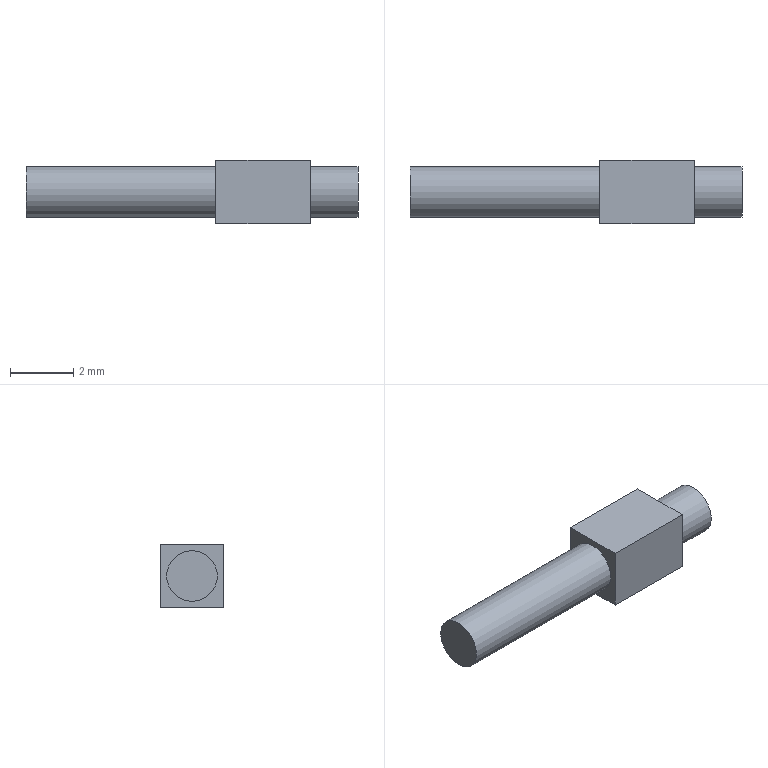Component | NX | MID_RECT_2_CIRC_2 | 1 solid | 10 faces | box 10.5 x 2 x 2 mm | volume 27 mm3 | plane 8 | cylinder 2 | commonest cylinder face diameters 1.6 x2
STEP:
#1=CARTESIAN_POINT('',(0.,0.,0.));
#2=DIRECTION('',(0.,0.,1.));
#3=DIRECTION('',(1.,0.,0.));
#4=AXIS2_PLACEMENT_3D('',#1,#2,#3);
#5=CARTESIAN_POINT('',(15.5,22.225,29.));
#6=VERTEX_POINT('',#5);
#7=CARTESIAN_POINT('',(18.5,22.225,29.));
#8=VERTEX_POINT('',#7);
#9=CARTESIAN_POINT('',(15.5,22.225,29.));
#10=DIRECTION('',(1.,-0.,0.));
#11=VECTOR('',#10,1.);
#12=LINE('',#9,#11);
#13=CARTESIAN_POINT('',(15.5,22.225,31.));
#14=DIRECTION('',(0.,1.,0.));
#15=DIRECTION('',(-1.,0.,0.));
#16=AXIS2_PLACEMENT_3D('',#13,#14,#15);
#17=PLANE('',#16);
#18=CARTESIAN_POINT('',(0.,-2.));
#19=DIRECTION('',(-1.,0.));
#20=VECTOR('',#19,1.);
#21=LINE('',#18,#20);
#22=(GEOMETRIC_REPRESENTATION_CONTEXT(2)PARAMETRIC_REPRESENTATION_CONTEXT()REPRESENTATION_CONTEXT('',''));
#23=DEFINITIONAL_REPRESENTATION('',(#21),#22);
#24=PCURVE('',#17,#23);
#25=CARTESIAN_POINT('',(17.,23.225,29.));
#26=DIRECTION('',(0.,0.,1.));
#27=DIRECTION('',(1.,0.,0.));
#28=AXIS2_PLACEMENT_3D('',#25,#26,#27);
#29=PLANE('',#28);
#30=CARTESIAN_POINT('',(-1.5,-1.));
#31=DIRECTION('',(1.,-0.));
#32=VECTOR('',#31,1.);
#33=LINE('',#30,#32);
#34=(GEOMETRIC_REPRESENTATION_CONTEXT(2)PARAMETRIC_REPRESENTATION_CONTEXT()REPRESENTATION_CONTEXT('',''));
#35=DEFINITIONAL_REPRESENTATION('',(#33),#34);
#36=PCURVE('',#29,#35);
#37=SURFACE_CURVE('',#12,(#24,#36),.PCURVE_S1.);
#38=EDGE_CURVE('',#6,#8,#37,.T.);
#39=ORIENTED_EDGE('',*,*,#38,.T.);
#40=CARTESIAN_POINT('',(18.5,22.225,31.));
#41=VERTEX_POINT('',#40);
#42=CARTESIAN_POINT('',(18.5,22.225,31.));
#43=DIRECTION('',(0.,0.,-1.));
#44=VECTOR('',#43,1.);
#45=LINE('',#42,#44);
#46=CARTESIAN_POINT('',(-3.,0.));
#47=DIRECTION('',(0.,-1.));
#48=VECTOR('',#47,1.);
#49=LINE('',#46,#48);
#50=(GEOMETRIC_REPRESENTATION_CONTEXT(2)PARAMETRIC_REPRESENTATION_CONTEXT()REPRESENTATION_CONTEXT('',''));
#51=DEFINITIONAL_REPRESENTATION('',(#49),#50);
#52=PCURVE('',#17,#51);
#53=CARTESIAN_POINT('',(18.5,22.225,31.));
#54=DIRECTION('',(-1.,0.,0.));
#55=DIRECTION('',(0.,0.,1.));
#56=AXIS2_PLACEMENT_3D('',#53,#54,#55);
#57=PLANE('',#56);
#58=CARTESIAN_POINT('',(0.,0.));
#59=DIRECTION('',(-1.,0.));
#60=VECTOR('',#59,1.);
#61=LINE('',#58,#60);
#62=(GEOMETRIC_REPRESENTATION_CONTEXT(2)PARAMETRIC_REPRESENTATION_CONTEXT()REPRESENTATION_CONTEXT('',''));
#63=DEFINITIONAL_REPRESENTATION('',(#61),#62);
#64=PCURVE('',#57,#63);
#65=SURFACE_CURVE('',#45,(#52,#64),.PCURVE_S1.);
#66=EDGE_CURVE('',#41,#8,#65,.T.);
#67=ORIENTED_EDGE('',*,*,#66,.F.);
#68=CARTESIAN_POINT('',(15.5,22.225,31.));
#69=VERTEX_POINT('',#68);
#70=CARTESIAN_POINT('',(15.5,22.225,31.));
#71=DIRECTION('',(1.,-0.,0.));
#72=VECTOR('',#71,1.);
#73=LINE('',#70,#72);
#74=CARTESIAN_POINT('',(0.,0.));
#75=DIRECTION('',(-1.,0.));
#76=VECTOR('',#75,1.);
#77=LINE('',#74,#76);
#78=(GEOMETRIC_REPRESENTATION_CONTEXT(2)PARAMETRIC_REPRESENTATION_CONTEXT()REPRESENTATION_CONTEXT('',''));
#79=DEFINITIONAL_REPRESENTATION('',(#77),#78);
#80=PCURVE('',#17,#79);
#81=CARTESIAN_POINT('',(17.,23.225,31.));
#82=DIRECTION('',(0.,0.,1.));
#83=DIRECTION('',(1.,0.,0.));
#84=AXIS2_PLACEMENT_3D('',#81,#82,#83);
#85=PLANE('',#84);
#86=CARTESIAN_POINT('',(-1.5,-1.));
#87=DIRECTION('',(1.,-0.));
#88=VECTOR('',#87,1.);
#89=LINE('',#86,#88);
#90=(GEOMETRIC_REPRESENTATION_CONTEXT(2)PARAMETRIC_REPRESENTATION_CONTEXT()REPRESENTATION_CONTEXT('',''));
#91=DEFINITIONAL_REPRESENTATION('',(#89),#90);
#92=PCURVE('',#85,#91);
#93=SURFACE_CURVE('',#73,(#80,#92),.PCURVE_S1.);
#94=EDGE_CURVE('',#69,#41,#93,.T.);
#95=ORIENTED_EDGE('',*,*,#94,.F.);
#96=CARTESIAN_POINT('',(15.5,22.225,31.));
#97=DIRECTION('',(0.,0.,-1.));
#98=VECTOR('',#97,1.);
#99=LINE('',#96,#98);
#100=CARTESIAN_POINT('',(0.,0.));
#101=DIRECTION('',(0.,-1.));
#102=VECTOR('',#101,1.);
#103=LINE('',#100,#102);
#104=(GEOMETRIC_REPRESENTATION_CONTEXT(2)PARAMETRIC_REPRESENTATION_CONTEXT()REPRESENTATION_CONTEXT('',''));
#105=DEFINITIONAL_REPRESENTATION('',(#103),#104);
#106=PCURVE('',#17,#105);
#107=CARTESIAN_POINT('',(15.5,24.225,31.));
#108=DIRECTION('',(1.,0.,0.));
#109=DIRECTION('',(0.,0.,-1.));
#110=AXIS2_PLACEMENT_3D('',#107,#108,#109);
#111=PLANE('',#110);
#112=CARTESIAN_POINT('',(0.,-2.));
#113=DIRECTION('',(1.,0.));
#114=VECTOR('',#113,1.);
#115=LINE('',#112,#114);
#116=(GEOMETRIC_REPRESENTATION_CONTEXT(2)PARAMETRIC_REPRESENTATION_CONTEXT()REPRESENTATION_CONTEXT('',''));
#117=DEFINITIONAL_REPRESENTATION('',(#115),#116);
#118=PCURVE('',#111,#117);
#119=SURFACE_CURVE('',#99,(#106,#118),.PCURVE_S1.);
#120=EDGE_CURVE('',#69,#6,#119,.T.);
#121=ORIENTED_EDGE('',*,*,#120,.T.);
#122=EDGE_LOOP('',(#39,#67,#95,#121));
#123=FACE_BOUND('',#122,.T.);
#124=ADVANCED_FACE('',(#123),#17,.F.);
#125=CARTESIAN_POINT('',(18.5,23.225,30.8));
#126=VERTEX_POINT('',#125);
#127=CARTESIAN_POINT('',(18.5,23.225,30.));
#128=DIRECTION('',(1.,0.,0.));
#129=DIRECTION('',(0.,0.,1.));
#130=AXIS2_PLACEMENT_3D('',#127,#128,#129);
#131=CIRCLE('',#130,0.8);
#132=CARTESIAN_POINT('',(-0.2,1.));
#133=CARTESIAN_POINT('',(-0.2,-0.3856));
#134=CARTESIAN_POINT('',(-1.4,0.3072));
#135=CARTESIAN_POINT('',(-2.6,1.));
#136=CARTESIAN_POINT('',(-1.4,1.693));
#137=CARTESIAN_POINT('',(-0.2,2.386));
#138=CARTESIAN_POINT('',(-0.2,1.));
#139=(BOUNDED_CURVE()B_SPLINE_CURVE(2,(#132,#133,#134,#135,#136,#137,#138),.UNSPECIFIED.,.T.,.F.)B_SPLINE_CURVE_WITH_KNOTS((1,2,2,2,2,1),(-2.094,0.,2.094,4.189,6.283,8.378),.UNSPECIFIED.)CURVE()GEOMETRIC_REPRESENTATION_ITEM()RATIONAL_B_SPLINE_CURVE((1.,0.5,1.,0.5,1.,0.5,1.))REPRESENTATION_ITEM(''));
#140=(GEOMETRIC_REPRESENTATION_CONTEXT(2)PARAMETRIC_REPRESENTATION_CONTEXT()REPRESENTATION_CONTEXT('',''));
#141=DEFINITIONAL_REPRESENTATION('',(#139),#140);
#142=PCURVE('',#57,#141);
#143=CARTESIAN_POINT('',(9.5,23.225,30.));
#144=DIRECTION('',(1.,0.,0.));
#145=DIRECTION('',(0.,0.,-1.));
#146=AXIS2_PLACEMENT_3D('',#143,#144,#145);
#147=CYLINDRICAL_SURFACE('',#146,0.8);
#148=CARTESIAN_POINT('',(3.142,9.));
#149=DIRECTION('',(1.,0.));
#150=VECTOR('',#149,1.);
#151=LINE('',#148,#150);
#152=(GEOMETRIC_REPRESENTATION_CONTEXT(2)PARAMETRIC_REPRESENTATION_CONTEXT()REPRESENTATION_CONTEXT('',''));
#153=DEFINITIONAL_REPRESENTATION('',(#151),#152);
#154=PCURVE('',#147,#153);
#155=SURFACE_CURVE('',#131,(#142,#154),.PCURVE_S1.);
#156=EDGE_CURVE('',#126,#126,#155,.T.);
#157=ORIENTED_EDGE('',*,*,#156,.F.);
#158=EDGE_LOOP('',(#157));
#159=FACE_BOUND('',#158,.T.);
#160=CARTESIAN_POINT('',(18.5,24.225,29.));
#161=VERTEX_POINT('',#160);
#162=CARTESIAN_POINT('',(18.5,22.225,29.));
#163=DIRECTION('',(0.,1.,0.));
#164=VECTOR('',#163,1.);
#165=LINE('',#162,#164);
#166=CARTESIAN_POINT('',(-2.,0.));
#167=DIRECTION('',(0.,1.));
#168=VECTOR('',#167,1.);
#169=LINE('',#166,#168);
#170=(GEOMETRIC_REPRESENTATION_CONTEXT(2)PARAMETRIC_REPRESENTATION_CONTEXT()REPRESENTATION_CONTEXT('',''));
#171=DEFINITIONAL_REPRESENTATION('',(#169),#170);
#172=PCURVE('',#57,#171);
#173=CARTESIAN_POINT('',(1.5,-1.));
#174=DIRECTION('',(0.,1.));
#175=VECTOR('',#174,1.);
#176=LINE('',#173,#175);
#177=(GEOMETRIC_REPRESENTATION_CONTEXT(2)PARAMETRIC_REPRESENTATION_CONTEXT()REPRESENTATION_CONTEXT('',''));
#178=DEFINITIONAL_REPRESENTATION('',(#176),#177);
#179=PCURVE('',#29,#178);
#180=SURFACE_CURVE('',#165,(#172,#179),.PCURVE_S1.);
#181=EDGE_CURVE('',#8,#161,#180,.T.);
#182=ORIENTED_EDGE('',*,*,#181,.T.);
#183=CARTESIAN_POINT('',(18.5,24.225,31.));
#184=VERTEX_POINT('',#183);
#185=CARTESIAN_POINT('',(18.5,24.225,31.));
#186=DIRECTION('',(0.,0.,-1.));
#187=VECTOR('',#186,1.);
#188=LINE('',#185,#187);
#189=CARTESIAN_POINT('',(0.,2.));
#190=DIRECTION('',(-1.,0.));
#191=VECTOR('',#190,1.);
#192=LINE('',#189,#191);
#193=(GEOMETRIC_REPRESENTATION_CONTEXT(2)PARAMETRIC_REPRESENTATION_CONTEXT()REPRESENTATION_CONTEXT('',''));
#194=DEFINITIONAL_REPRESENTATION('',(#192),#193);
#195=PCURVE('',#57,#194);
#196=CARTESIAN_POINT('',(18.5,24.225,31.));
#197=DIRECTION('',(-0.,-1.,0.));
#198=DIRECTION('',(1.,-0.,0.));
#199=AXIS2_PLACEMENT_3D('',#196,#197,#198);
#200=PLANE('',#199);
#201=CARTESIAN_POINT('',(0.,0.));
#202=DIRECTION('',(0.,-1.));
#203=VECTOR('',#202,1.);
#204=LINE('',#201,#203);
#205=(GEOMETRIC_REPRESENTATION_CONTEXT(2)PARAMETRIC_REPRESENTATION_CONTEXT()REPRESENTATION_CONTEXT('',''));
#206=DEFINITIONAL_REPRESENTATION('',(#204),#205);
#207=PCURVE('',#200,#206);
#208=SURFACE_CURVE('',#188,(#195,#207),.PCURVE_S1.);
#209=EDGE_CURVE('',#184,#161,#208,.T.);
#210=ORIENTED_EDGE('',*,*,#209,.F.);
#211=CARTESIAN_POINT('',(18.5,22.225,31.));
#212=DIRECTION('',(0.,1.,0.));
#213=VECTOR('',#212,1.);
#214=LINE('',#211,#213);
#215=CARTESIAN_POINT('',(0.,0.));
#216=DIRECTION('',(0.,1.));
#217=VECTOR('',#216,1.);
#218=LINE('',#215,#217);
#219=(GEOMETRIC_REPRESENTATION_CONTEXT(2)PARAMETRIC_REPRESENTATION_CONTEXT()REPRESENTATION_CONTEXT('',''));
#220=DEFINITIONAL_REPRESENTATION('',(#218),#219);
#221=PCURVE('',#57,#220);
#222=CARTESIAN_POINT('',(1.5,-1.));
#223=DIRECTION('',(0.,1.));
#224=VECTOR('',#223,1.);
#225=LINE('',#222,#224);
#226=(GEOMETRIC_REPRESENTATION_CONTEXT(2)PARAMETRIC_REPRESENTATION_CONTEXT()REPRESENTATION_CONTEXT('',''));
#227=DEFINITIONAL_REPRESENTATION('',(#225),#226);
#228=PCURVE('',#85,#227);
#229=SURFACE_CURVE('',#214,(#221,#228),.PCURVE_S1.);
#230=EDGE_CURVE('',#41,#184,#229,.T.);
#231=ORIENTED_EDGE('',*,*,#230,.F.);
#232=ORIENTED_EDGE('',*,*,#66,.T.);
#233=EDGE_LOOP('',(#182,#210,#231,#232));
#234=FACE_BOUND('',#233,.T.);
#235=ADVANCED_FACE('',(#159,#234),#57,.F.);
#236=CARTESIAN_POINT('',(15.5,24.225,29.));
#237=VERTEX_POINT('',#236);
#238=CARTESIAN_POINT('',(18.5,24.225,29.));
#239=DIRECTION('',(-1.,0.,0.));
#240=VECTOR('',#239,1.);
#241=LINE('',#238,#240);
#242=CARTESIAN_POINT('',(0.,-2.));
#243=DIRECTION('',(-1.,0.));
#244=VECTOR('',#243,1.);
#245=LINE('',#242,#244);
#246=(GEOMETRIC_REPRESENTATION_CONTEXT(2)PARAMETRIC_REPRESENTATION_CONTEXT()REPRESENTATION_CONTEXT('',''));
#247=DEFINITIONAL_REPRESENTATION('',(#245),#246);
#248=PCURVE('',#200,#247);
#249=CARTESIAN_POINT('',(1.5,1.));
#250=DIRECTION('',(-1.,0.));
#251=VECTOR('',#250,1.);
#252=LINE('',#249,#251);
#253=(GEOMETRIC_REPRESENTATION_CONTEXT(2)PARAMETRIC_REPRESENTATION_CONTEXT()REPRESENTATION_CONTEXT('',''));
#254=DEFINITIONAL_REPRESENTATION('',(#252),#253);
#255=PCURVE('',#29,#254);
#256=SURFACE_CURVE('',#241,(#248,#255),.PCURVE_S1.);
#257=EDGE_CURVE('',#161,#237,#256,.T.);
#258=ORIENTED_EDGE('',*,*,#257,.T.);
#259=CARTESIAN_POINT('',(15.5,24.225,31.));
#260=VERTEX_POINT('',#259);
#261=CARTESIAN_POINT('',(15.5,24.225,31.));
#262=DIRECTION('',(0.,0.,-1.));
#263=VECTOR('',#262,1.);
#264=LINE('',#261,#263);
#265=CARTESIAN_POINT('',(-3.,0.));
#266=DIRECTION('',(0.,-1.));
#267=VECTOR('',#266,1.);
#268=LINE('',#265,#267);
#269=(GEOMETRIC_REPRESENTATION_CONTEXT(2)PARAMETRIC_REPRESENTATION_CONTEXT()REPRESENTATION_CONTEXT('',''));
#270=DEFINITIONAL_REPRESENTATION('',(#268),#269);
#271=PCURVE('',#200,#270);
#272=CARTESIAN_POINT('',(0.,0.));
#273=DIRECTION('',(1.,0.));
#274=VECTOR('',#273,1.);
#275=LINE('',#272,#274);
#276=(GEOMETRIC_REPRESENTATION_CONTEXT(2)PARAMETRIC_REPRESENTATION_CONTEXT()REPRESENTATION_CONTEXT('',''));
#277=DEFINITIONAL_REPRESENTATION('',(#275),#276);
#278=PCURVE('',#111,#277);
#279=SURFACE_CURVE('',#264,(#271,#278),.PCURVE_S1.);
#280=EDGE_CURVE('',#260,#237,#279,.T.);
#281=ORIENTED_EDGE('',*,*,#280,.F.);
#282=CARTESIAN_POINT('',(18.5,24.225,31.));
#283=DIRECTION('',(-1.,0.,0.));
#284=VECTOR('',#283,1.);
#285=LINE('',#282,#284);
#286=CARTESIAN_POINT('',(0.,0.));
#287=DIRECTION('',(-1.,0.));
#288=VECTOR('',#287,1.);
#289=LINE('',#286,#288);
#290=(GEOMETRIC_REPRESENTATION_CONTEXT(2)PARAMETRIC_REPRESENTATION_CONTEXT()REPRESENTATION_CONTEXT('',''));
#291=DEFINITIONAL_REPRESENTATION('',(#289),#290);
#292=PCURVE('',#200,#291);
#293=CARTESIAN_POINT('',(1.5,1.));
#294=DIRECTION('',(-1.,0.));
#295=VECTOR('',#294,1.);
#296=LINE('',#293,#295);
#297=(GEOMETRIC_REPRESENTATION_CONTEXT(2)PARAMETRIC_REPRESENTATION_CONTEXT()REPRESENTATION_CONTEXT('',''));
#298=DEFINITIONAL_REPRESENTATION('',(#296),#297);
#299=PCURVE('',#85,#298);
#300=SURFACE_CURVE('',#285,(#292,#299),.PCURVE_S1.);
#301=EDGE_CURVE('',#184,#260,#300,.T.);
#302=ORIENTED_EDGE('',*,*,#301,.F.);
#303=ORIENTED_EDGE('',*,*,#209,.T.);
#304=EDGE_LOOP('',(#258,#281,#302,#303));
#305=FACE_BOUND('',#304,.T.);
#306=ADVANCED_FACE('',(#305),#200,.F.);
#307=CARTESIAN_POINT('',(15.5,23.225,29.2));
#308=VERTEX_POINT('',#307);
#309=CARTESIAN_POINT('',(15.5,23.225,30.));
#310=DIRECTION('',(-1.,0.,0.));
#311=DIRECTION('',(0.,0.,-1.));
#312=AXIS2_PLACEMENT_3D('',#309,#310,#311);
#313=CIRCLE('',#312,0.8);
#314=CARTESIAN_POINT('',(1.8,-1.));
#315=CARTESIAN_POINT('',(1.8,-2.386));
#316=CARTESIAN_POINT('',(0.6,-1.693));
#317=CARTESIAN_POINT('',(-0.6,-1.));
#318=CARTESIAN_POINT('',(0.6,-0.3072));
#319=CARTESIAN_POINT('',(1.8,0.3856));
#320=CARTESIAN_POINT('',(1.8,-1.));
#321=(BOUNDED_CURVE()B_SPLINE_CURVE(2,(#314,#315,#316,#317,#318,#319,#320),.UNSPECIFIED.,.T.,.F.)B_SPLINE_CURVE_WITH_KNOTS((1,2,2,2,2,1),(-2.094,0.,2.094,4.189,6.283,8.378),.UNSPECIFIED.)CURVE()GEOMETRIC_REPRESENTATION_ITEM()RATIONAL_B_SPLINE_CURVE((1.,0.5,1.,0.5,1.,0.5,1.))REPRESENTATION_ITEM(''));
#322=(GEOMETRIC_REPRESENTATION_CONTEXT(2)PARAMETRIC_REPRESENTATION_CONTEXT()REPRESENTATION_CONTEXT('',''));
#323=DEFINITIONAL_REPRESENTATION('',(#321),#322);
#324=PCURVE('',#111,#323);
#325=CARTESIAN_POINT('',(9.5,23.225,30.));
#326=DIRECTION('',(1.,0.,0.));
#327=DIRECTION('',(0.,0.,-1.));
#328=AXIS2_PLACEMENT_3D('',#325,#326,#327);
#329=CYLINDRICAL_SURFACE('',#328,0.8);
#330=CARTESIAN_POINT('',(6.283,6.));
#331=DIRECTION('',(-1.,0.));
#332=VECTOR('',#331,1.);
#333=LINE('',#330,#332);
#334=(GEOMETRIC_REPRESENTATION_CONTEXT(2)PARAMETRIC_REPRESENTATION_CONTEXT()REPRESENTATION_CONTEXT('',''));
#335=DEFINITIONAL_REPRESENTATION('',(#333),#334);
#336=PCURVE('',#329,#335);
#337=SURFACE_CURVE('',#313,(#324,#336),.PCURVE_S1.);
#338=EDGE_CURVE('',#308,#308,#337,.T.);
#339=ORIENTED_EDGE('',*,*,#338,.F.);
#340=EDGE_LOOP('',(#339));
#341=FACE_BOUND('',#340,.T.);
#342=CARTESIAN_POINT('',(15.5,24.225,29.));
#343=DIRECTION('',(0.,-1.,0.));
#344=VECTOR('',#343,1.);
#345=LINE('',#342,#344);
#346=CARTESIAN_POINT('',(2.,0.));
#347=DIRECTION('',(0.,-1.));
#348=VECTOR('',#347,1.);
#349=LINE('',#346,#348);
#350=(GEOMETRIC_REPRESENTATION_CONTEXT(2)PARAMETRIC_REPRESENTATION_CONTEXT()REPRESENTATION_CONTEXT('',''));
#351=DEFINITIONAL_REPRESENTATION('',(#349),#350);
#352=PCURVE('',#111,#351);
#353=CARTESIAN_POINT('',(-1.5,1.));
#354=DIRECTION('',(0.,-1.));
#355=VECTOR('',#354,1.);
#356=LINE('',#353,#355);
#357=(GEOMETRIC_REPRESENTATION_CONTEXT(2)PARAMETRIC_REPRESENTATION_CONTEXT()REPRESENTATION_CONTEXT('',''));
#358=DEFINITIONAL_REPRESENTATION('',(#356),#357);
#359=PCURVE('',#29,#358);
#360=SURFACE_CURVE('',#345,(#352,#359),.PCURVE_S1.);
#361=EDGE_CURVE('',#237,#6,#360,.T.);
#362=ORIENTED_EDGE('',*,*,#361,.T.);
#363=ORIENTED_EDGE('',*,*,#120,.F.);
#364=CARTESIAN_POINT('',(15.5,24.225,31.));
#365=DIRECTION('',(0.,-1.,0.));
#366=VECTOR('',#365,1.);
#367=LINE('',#364,#366);
#368=CARTESIAN_POINT('',(0.,0.));
#369=DIRECTION('',(0.,-1.));
#370=VECTOR('',#369,1.);
#371=LINE('',#368,#370);
#372=(GEOMETRIC_REPRESENTATION_CONTEXT(2)PARAMETRIC_REPRESENTATION_CONTEXT()REPRESENTATION_CONTEXT('',''));
#373=DEFINITIONAL_REPRESENTATION('',(#371),#372);
#374=PCURVE('',#111,#373);
#375=CARTESIAN_POINT('',(-1.5,1.));
#376=DIRECTION('',(0.,-1.));
#377=VECTOR('',#376,1.);
#378=LINE('',#375,#377);
#379=(GEOMETRIC_REPRESENTATION_CONTEXT(2)PARAMETRIC_REPRESENTATION_CONTEXT()REPRESENTATION_CONTEXT('',''));
#380=DEFINITIONAL_REPRESENTATION('',(#378),#379);
#381=PCURVE('',#85,#380);
#382=SURFACE_CURVE('',#367,(#374,#381),.PCURVE_S1.);
#383=EDGE_CURVE('',#260,#69,#382,.T.);
#384=ORIENTED_EDGE('',*,*,#383,.F.);
#385=ORIENTED_EDGE('',*,*,#280,.T.);
#386=EDGE_LOOP('',(#362,#363,#384,#385));
#387=FACE_BOUND('',#386,.T.);
#388=ADVANCED_FACE('',(#341,#387),#111,.F.);
#389=ORIENTED_EDGE('',*,*,#94,.T.);
#390=ORIENTED_EDGE('',*,*,#230,.T.);
#391=ORIENTED_EDGE('',*,*,#301,.T.);
#392=ORIENTED_EDGE('',*,*,#383,.T.);
#393=EDGE_LOOP('',(#389,#390,#391,#392));
#394=FACE_BOUND('',#393,.T.);
#395=ADVANCED_FACE('',(#394),#85,.T.);
#396=ORIENTED_EDGE('',*,*,#38,.F.);
#397=ORIENTED_EDGE('',*,*,#361,.F.);
#398=ORIENTED_EDGE('',*,*,#257,.F.);
#399=ORIENTED_EDGE('',*,*,#181,.F.);
#400=EDGE_LOOP('',(#396,#397,#398,#399));
#401=FACE_BOUND('',#400,.T.);
#402=ADVANCED_FACE('',(#401),#29,.F.);
#403=CARTESIAN_POINT('',(9.5,23.225,30.8));
#404=VERTEX_POINT('',#403);
#405=CARTESIAN_POINT('',(9.5,23.225,29.2));
#406=VERTEX_POINT('',#405);
#407=CARTESIAN_POINT('',(9.5,23.225,30.));
#408=DIRECTION('',(-1.,0.,0.));
#409=DIRECTION('',(0.,0.,1.));
#410=AXIS2_PLACEMENT_3D('',#407,#408,#409);
#411=CIRCLE('',#410,0.8);
#412=CARTESIAN_POINT('',(9.5,23.225,30.));
#413=DIRECTION('',(-1.,0.,0.));
#414=DIRECTION('',(0.,0.,1.));
#415=AXIS2_PLACEMENT_3D('',#412,#413,#414);
#416=PLANE('',#415);
#417=CARTESIAN_POINT('',(0.,0.));
#418=DIRECTION('',(1.,0.));
#419=AXIS2_PLACEMENT_2D('',#417,#418);
#420=CIRCLE('',#419,0.8);
#421=(GEOMETRIC_REPRESENTATION_CONTEXT(2)PARAMETRIC_REPRESENTATION_CONTEXT()REPRESENTATION_CONTEXT('',''));
#422=DEFINITIONAL_REPRESENTATION('',(#420),#421);
#423=PCURVE('',#416,#422);
#424=CARTESIAN_POINT('',(3.142,0.));
#425=DIRECTION('',(-1.,0.));
#426=VECTOR('',#425,1.);
#427=LINE('',#424,#426);
#428=(GEOMETRIC_REPRESENTATION_CONTEXT(2)PARAMETRIC_REPRESENTATION_CONTEXT()REPRESENTATION_CONTEXT('',''));
#429=DEFINITIONAL_REPRESENTATION('',(#427),#428);
#430=PCURVE('',#329,#429);
#431=SURFACE_CURVE('',#411,(#423,#430),.PCURVE_S1.);
#432=EDGE_CURVE('',#404,#406,#431,.T.);
#433=ORIENTED_EDGE('',*,*,#432,.T.);
#434=CARTESIAN_POINT('',(9.5,23.225,30.));
#435=DIRECTION('',(-1.,0.,0.));
#436=DIRECTION('',(0.,0.,1.));
#437=AXIS2_PLACEMENT_3D('',#434,#435,#436);
#438=CIRCLE('',#437,0.8);
#439=CARTESIAN_POINT('',(0.,0.));
#440=DIRECTION('',(1.,0.));
#441=AXIS2_PLACEMENT_2D('',#439,#440);
#442=CIRCLE('',#441,0.8);
#443=(GEOMETRIC_REPRESENTATION_CONTEXT(2)PARAMETRIC_REPRESENTATION_CONTEXT()REPRESENTATION_CONTEXT('',''));
#444=DEFINITIONAL_REPRESENTATION('',(#442),#443);
#445=PCURVE('',#416,#444);
#446=CARTESIAN_POINT('',(9.425,0.));
#447=DIRECTION('',(-1.,0.));
#448=VECTOR('',#447,1.);
#449=LINE('',#446,#448);
#450=(GEOMETRIC_REPRESENTATION_CONTEXT(2)PARAMETRIC_REPRESENTATION_CONTEXT()REPRESENTATION_CONTEXT('',''));
#451=DEFINITIONAL_REPRESENTATION('',(#449),#450);
#452=PCURVE('',#329,#451);
#453=SURFACE_CURVE('',#438,(#445,#452),.PCURVE_S1.);
#454=EDGE_CURVE('',#406,#404,#453,.T.);
#455=ORIENTED_EDGE('',*,*,#454,.T.);
#456=EDGE_LOOP('',(#433,#455));
#457=FACE_BOUND('',#456,.T.);
#458=ADVANCED_FACE('',(#457),#416,.T.);
#459=ORIENTED_EDGE('',*,*,#454,.F.);
#460=CARTESIAN_POINT('',(9.5,23.225,29.2));
#461=CARTESIAN_POINT('',(15.5,23.225,29.2));
#462=B_SPLINE_CURVE_WITH_KNOTS('',1,(#460,#461),.UNSPECIFIED.,.F.,.F.,(2,2),(0.,6.),.PIECEWISE_BEZIER_KNOTS.);
#463=CARTESIAN_POINT('',(6.283,0.));
#464=DIRECTION('',(0.,1.));
#465=VECTOR('',#464,1.);
#466=LINE('',#463,#465);
#467=(GEOMETRIC_REPRESENTATION_CONTEXT(2)PARAMETRIC_REPRESENTATION_CONTEXT()REPRESENTATION_CONTEXT('',''));
#468=DEFINITIONAL_REPRESENTATION('',(#466),#467);
#469=PCURVE('',#329,#468);
#470=CARTESIAN_POINT('',(0.,0.));
#471=DIRECTION('',(0.,1.));
#472=VECTOR('',#471,1.);
#473=LINE('',#470,#472);
#474=(GEOMETRIC_REPRESENTATION_CONTEXT(2)PARAMETRIC_REPRESENTATION_CONTEXT()REPRESENTATION_CONTEXT('',''));
#475=DEFINITIONAL_REPRESENTATION('',(#473),#474);
#476=PCURVE('',#329,#475);
#477=SEAM_CURVE('',#462,(#469,#476),.PCURVE_S1.);
#478=EDGE_CURVE('',#406,#308,#477,.T.);
#479=ORIENTED_EDGE('',*,*,#478,.T.);
#480=ORIENTED_EDGE('',*,*,#338,.T.);
#481=ORIENTED_EDGE('',*,*,#478,.F.);
#482=ORIENTED_EDGE('',*,*,#432,.F.);
#483=EDGE_LOOP('',(#459,#479,#480,#481,#482));
#484=FACE_BOUND('',#483,.T.);
#485=ADVANCED_FACE('',(#484),#329,.T.);
#486=CARTESIAN_POINT('',(20.,23.225,30.8));
#487=VERTEX_POINT('',#486);
#488=CARTESIAN_POINT('',(20.,23.225,30.));
#489=DIRECTION('',(-1.,0.,0.));
#490=DIRECTION('',(0.,0.,1.));
#491=AXIS2_PLACEMENT_3D('',#488,#489,#490);
#492=CIRCLE('',#491,0.8);
#493=CARTESIAN_POINT('',(9.425,10.5));
#494=DIRECTION('',(-1.,0.));
#495=VECTOR('',#494,1.);
#496=LINE('',#493,#495);
#497=(GEOMETRIC_REPRESENTATION_CONTEXT(2)PARAMETRIC_REPRESENTATION_CONTEXT()REPRESENTATION_CONTEXT('',''));
#498=DEFINITIONAL_REPRESENTATION('',(#496),#497);
#499=PCURVE('',#147,#498);
#500=CARTESIAN_POINT('',(20.,23.225,30.));
#501=DIRECTION('',(-1.,0.,0.));
#502=DIRECTION('',(0.,0.,1.));
#503=AXIS2_PLACEMENT_3D('',#500,#501,#502);
#504=PLANE('',#503);
#505=CARTESIAN_POINT('',(0.,0.));
#506=DIRECTION('',(1.,0.));
#507=AXIS2_PLACEMENT_2D('',#505,#506);
#508=CIRCLE('',#507,0.8);
#509=(GEOMETRIC_REPRESENTATION_CONTEXT(2)PARAMETRIC_REPRESENTATION_CONTEXT()REPRESENTATION_CONTEXT('',''));
#510=DEFINITIONAL_REPRESENTATION('',(#508),#509);
#511=PCURVE('',#504,#510);
#512=SURFACE_CURVE('',#492,(#499,#511),.PCURVE_S1.);
#513=EDGE_CURVE('',#487,#487,#512,.T.);
#514=ORIENTED_EDGE('',*,*,#513,.T.);
#515=CARTESIAN_POINT('',(18.5,23.225,30.8));
#516=CARTESIAN_POINT('',(20.,23.225,30.8));
#517=B_SPLINE_CURVE_WITH_KNOTS('',1,(#515,#516),.UNSPECIFIED.,.F.,.F.,(2,2),(9.,10.5),.PIECEWISE_BEZIER_KNOTS.);
#518=CARTESIAN_POINT('',(3.142,0.));
#519=DIRECTION('',(0.,1.));
#520=VECTOR('',#519,1.);
#521=LINE('',#518,#520);
#522=(GEOMETRIC_REPRESENTATION_CONTEXT(2)PARAMETRIC_REPRESENTATION_CONTEXT()REPRESENTATION_CONTEXT('',''));
#523=DEFINITIONAL_REPRESENTATION('',(#521),#522);
#524=PCURVE('',#147,#523);
#525=CARTESIAN_POINT('',(9.425,0.));
#526=DIRECTION('',(0.,1.));
#527=VECTOR('',#526,1.);
#528=LINE('',#525,#527);
#529=(GEOMETRIC_REPRESENTATION_CONTEXT(2)PARAMETRIC_REPRESENTATION_CONTEXT()REPRESENTATION_CONTEXT('',''));
#530=DEFINITIONAL_REPRESENTATION('',(#528),#529);
#531=PCURVE('',#147,#530);
#532=SEAM_CURVE('',#517,(#524,#531),.PCURVE_S1.);
#533=EDGE_CURVE('',#126,#487,#532,.T.);
#534=ORIENTED_EDGE('',*,*,#533,.F.);
#535=ORIENTED_EDGE('',*,*,#156,.T.);
#536=ORIENTED_EDGE('',*,*,#533,.T.);
#537=EDGE_LOOP('',(#514,#534,#535,#536));
#538=FACE_BOUND('',#537,.T.);
#539=ADVANCED_FACE('',(#538),#147,.T.);
#540=ORIENTED_EDGE('',*,*,#513,.F.);
#541=EDGE_LOOP('',(#540));
#542=FACE_BOUND('',#541,.T.);
#543=ADVANCED_FACE('',(#542),#504,.F.);
#544=CLOSED_SHELL('',(#124,#235,#306,#388,#395,#402,#458,#485,#539,#543));
#545=MANIFOLD_SOLID_BREP('',#544);
#546=(LENGTH_UNIT()NAMED_UNIT(*)SI_UNIT(.MILLI.,.METRE.));
#547=UNCERTAINTY_MEASURE_WITH_UNIT(LENGTH_MEASURE(0.000002),#546,'','');
#548=(NAMED_UNIT(*)PLANE_ANGLE_UNIT()SI_UNIT($,.RADIAN.));
#549=(NAMED_UNIT(*)SI_UNIT($,.STERADIAN.)SOLID_ANGLE_UNIT());
#550=(GEOMETRIC_REPRESENTATION_CONTEXT(3)GLOBAL_UNCERTAINTY_ASSIGNED_CONTEXT((#547))GLOBAL_UNIT_ASSIGNED_CONTEXT((#546,#548,#549))REPRESENTATION_CONTEXT('',''));
#551=ADVANCED_BREP_SHAPE_REPRESENTATION('',(#4,#545),#550);